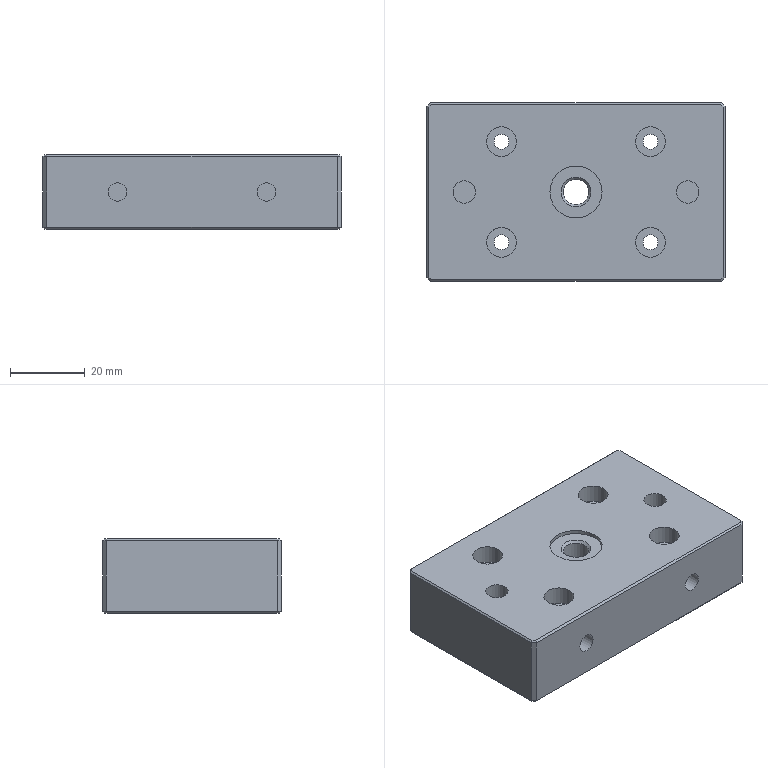Component | NX | ROBOT_CONN_PLATE | 1 solid | 65 faces | volume 72833 mm3 | plane 39 | cylinder 20 | cone 6 | commonest cylinder face diameters 8 x4 4 x4 5 x4 6 x2 6.5 x2 2.5 x2 14 x1 6.8 x1